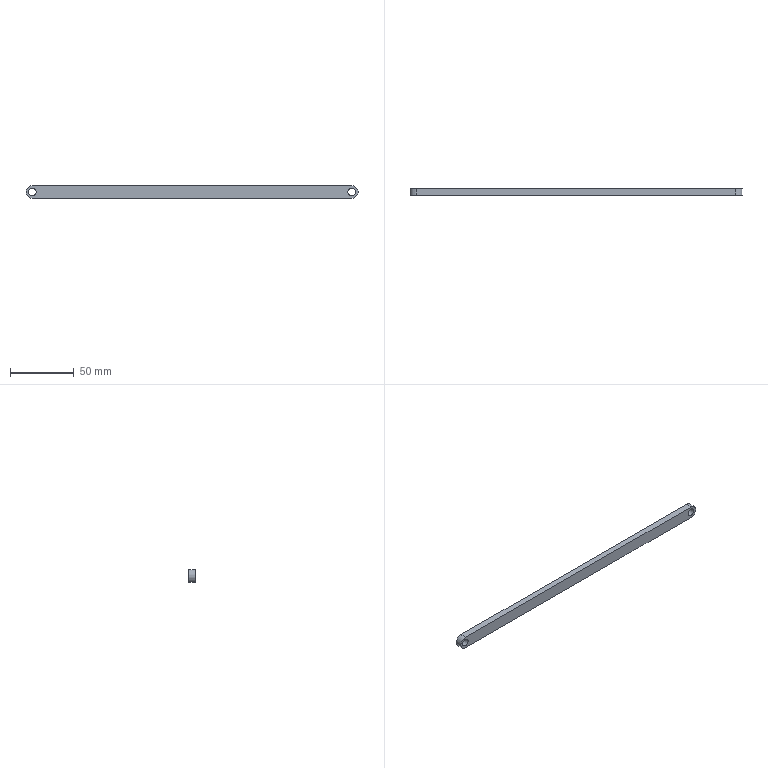Component | NX | 250 | 1 solid | 8 faces | box 260 x 5 x 10 mm | volume 12617 mm3 | plane 4 | cylinder 4 | commonest cylinder face diameters 10 x2 5.929 x2
STEP:
#1=CARTESIAN_POINT('',(0.,0.,0.));
#2=DIRECTION('',(0.,0.,1.));
#3=DIRECTION('',(1.,0.,0.));
#4=AXIS2_PLACEMENT_3D('',#1,#2,#3);
#5=CARTESIAN_POINT('',(-504.719,50.95,64.918));
#6=VERTEX_POINT('',#5);
#7=CARTESIAN_POINT('',(-254.719,50.95,64.918));
#8=VERTEX_POINT('',#7);
#9=CARTESIAN_POINT('',(-504.719,50.95,64.918));
#10=DIRECTION('',(1.,0.,-0.));
#11=VECTOR('',#10,1.);
#12=LINE('',#9,#11);
#13=CARTESIAN_POINT('',(-504.719,45.95,64.918));
#14=DIRECTION('',(0.,0.,1.));
#15=DIRECTION('',(1.,0.,-0.));
#16=AXIS2_PLACEMENT_3D('',#13,#14,#15);
#17=PLANE('',#16);
#18=CARTESIAN_POINT('',(0.,5.));
#19=DIRECTION('',(1.,0.));
#20=VECTOR('',#19,1.);
#21=LINE('',#18,#20);
#22=(GEOMETRIC_REPRESENTATION_CONTEXT(2)PARAMETRIC_REPRESENTATION_CONTEXT()REPRESENTATION_CONTEXT('',''));
#23=DEFINITIONAL_REPRESENTATION('',(#21),#22);
#24=PCURVE('',#17,#23);
#25=CARTESIAN_POINT('',(-254.719,50.95,59.918));
#26=DIRECTION('',(0.,1.,0.));
#27=DIRECTION('',(0.,0.,1.));
#28=AXIS2_PLACEMENT_3D('',#25,#26,#27);
#29=PLANE('',#28);
#30=CARTESIAN_POINT('',(5.,-250.));
#31=DIRECTION('',(-0.,1.));
#32=VECTOR('',#31,1.);
#33=LINE('',#30,#32);
#34=(GEOMETRIC_REPRESENTATION_CONTEXT(2)PARAMETRIC_REPRESENTATION_CONTEXT()REPRESENTATION_CONTEXT('',''));
#35=DEFINITIONAL_REPRESENTATION('',(#33),#34);
#36=PCURVE('',#29,#35);
#37=SURFACE_CURVE('',#12,(#24,#36),.PCURVE_S1.);
#38=EDGE_CURVE('',#6,#8,#37,.T.);
#39=ORIENTED_EDGE('',*,*,#38,.F.);
#40=CARTESIAN_POINT('',(-504.719,45.95,64.918));
#41=VERTEX_POINT('',#40);
#42=CARTESIAN_POINT('',(-504.719,45.95,64.918));
#43=DIRECTION('',(0.,1.,0.));
#44=VECTOR('',#43,1.);
#45=LINE('',#42,#44);
#46=CARTESIAN_POINT('',(0.,0.));
#47=DIRECTION('',(0.,1.));
#48=VECTOR('',#47,1.);
#49=LINE('',#46,#48);
#50=(GEOMETRIC_REPRESENTATION_CONTEXT(2)PARAMETRIC_REPRESENTATION_CONTEXT()REPRESENTATION_CONTEXT('',''));
#51=DEFINITIONAL_REPRESENTATION('',(#49),#50);
#52=PCURVE('',#17,#51);
#53=CARTESIAN_POINT('',(-504.719,45.95,59.918));
#54=DIRECTION('',(0.,1.,0.));
#55=DIRECTION('',(0.,0.,1.));
#56=AXIS2_PLACEMENT_3D('',#53,#54,#55);
#57=CYLINDRICAL_SURFACE('',#56,5.);
#58=CARTESIAN_POINT('',(6.283,0.));
#59=DIRECTION('',(0.,1.));
#60=VECTOR('',#59,1.);
#61=LINE('',#58,#60);
#62=(GEOMETRIC_REPRESENTATION_CONTEXT(2)PARAMETRIC_REPRESENTATION_CONTEXT()REPRESENTATION_CONTEXT('',''));
#63=DEFINITIONAL_REPRESENTATION('',(#61),#62);
#64=PCURVE('',#57,#63);
#65=SURFACE_CURVE('',#45,(#52,#64),.PCURVE_S1.);
#66=EDGE_CURVE('',#41,#6,#65,.T.);
#67=ORIENTED_EDGE('',*,*,#66,.F.);
#68=CARTESIAN_POINT('',(-254.719,45.95,64.918));
#69=VERTEX_POINT('',#68);
#70=CARTESIAN_POINT('',(-504.719,45.95,64.918));
#71=DIRECTION('',(1.,0.,-0.));
#72=VECTOR('',#71,1.);
#73=LINE('',#70,#72);
#74=CARTESIAN_POINT('',(0.,0.));
#75=DIRECTION('',(1.,0.));
#76=VECTOR('',#75,1.);
#77=LINE('',#74,#76);
#78=(GEOMETRIC_REPRESENTATION_CONTEXT(2)PARAMETRIC_REPRESENTATION_CONTEXT()REPRESENTATION_CONTEXT('',''));
#79=DEFINITIONAL_REPRESENTATION('',(#77),#78);
#80=PCURVE('',#17,#79);
#81=CARTESIAN_POINT('',(-254.719,45.95,59.918));
#82=DIRECTION('',(0.,1.,0.));
#83=DIRECTION('',(0.,0.,1.));
#84=AXIS2_PLACEMENT_3D('',#81,#82,#83);
#85=PLANE('',#84);
#86=CARTESIAN_POINT('',(5.,-250.));
#87=DIRECTION('',(-0.,1.));
#88=VECTOR('',#87,1.);
#89=LINE('',#86,#88);
#90=(GEOMETRIC_REPRESENTATION_CONTEXT(2)PARAMETRIC_REPRESENTATION_CONTEXT()REPRESENTATION_CONTEXT('',''));
#91=DEFINITIONAL_REPRESENTATION('',(#89),#90);
#92=PCURVE('',#85,#91);
#93=SURFACE_CURVE('',#73,(#80,#92),.PCURVE_S1.);
#94=EDGE_CURVE('',#41,#69,#93,.T.);
#95=ORIENTED_EDGE('',*,*,#94,.T.);
#96=CARTESIAN_POINT('',(-254.719,45.95,64.918));
#97=DIRECTION('',(0.,1.,0.));
#98=VECTOR('',#97,1.);
#99=LINE('',#96,#98);
#100=CARTESIAN_POINT('',(250.,0.));
#101=DIRECTION('',(0.,1.));
#102=VECTOR('',#101,1.);
#103=LINE('',#100,#102);
#104=(GEOMETRIC_REPRESENTATION_CONTEXT(2)PARAMETRIC_REPRESENTATION_CONTEXT()REPRESENTATION_CONTEXT('',''));
#105=DEFINITIONAL_REPRESENTATION('',(#103),#104);
#106=PCURVE('',#17,#105);
#107=CARTESIAN_POINT('',(-254.719,45.95,59.918));
#108=DIRECTION('',(0.,1.,0.));
#109=DIRECTION('',(0.,0.,1.));
#110=AXIS2_PLACEMENT_3D('',#107,#108,#109);
#111=CYLINDRICAL_SURFACE('',#110,5.);
#112=CARTESIAN_POINT('',(0.,0.));
#113=DIRECTION('',(0.,1.));
#114=VECTOR('',#113,1.);
#115=LINE('',#112,#114);
#116=(GEOMETRIC_REPRESENTATION_CONTEXT(2)PARAMETRIC_REPRESENTATION_CONTEXT()REPRESENTATION_CONTEXT('',''));
#117=DEFINITIONAL_REPRESENTATION('',(#115),#116);
#118=PCURVE('',#111,#117);
#119=SURFACE_CURVE('',#99,(#106,#118),.PCURVE_S1.);
#120=EDGE_CURVE('',#69,#8,#119,.T.);
#121=ORIENTED_EDGE('',*,*,#120,.T.);
#122=EDGE_LOOP('',(#39,#67,#95,#121));
#123=FACE_BOUND('',#122,.T.);
#124=ADVANCED_FACE('',(#123),#17,.T.);
#125=CARTESIAN_POINT('',(-254.719,50.95,54.918));
#126=VERTEX_POINT('',#125);
#127=CARTESIAN_POINT('',(-254.719,50.95,59.918));
#128=DIRECTION('',(0.,1.,0.));
#129=DIRECTION('',(0.,0.,1.));
#130=AXIS2_PLACEMENT_3D('',#127,#128,#129);
#131=CIRCLE('',#130,5.);
#132=CARTESIAN_POINT('',(0.,5.));
#133=DIRECTION('',(1.,0.));
#134=VECTOR('',#133,1.);
#135=LINE('',#132,#134);
#136=(GEOMETRIC_REPRESENTATION_CONTEXT(2)PARAMETRIC_REPRESENTATION_CONTEXT()REPRESENTATION_CONTEXT('',''));
#137=DEFINITIONAL_REPRESENTATION('',(#135),#136);
#138=PCURVE('',#111,#137);
#139=CARTESIAN_POINT('',(0.,0.));
#140=DIRECTION('',(1.,0.));
#141=AXIS2_PLACEMENT_2D('',#139,#140);
#142=CIRCLE('',#141,5.);
#143=(GEOMETRIC_REPRESENTATION_CONTEXT(2)PARAMETRIC_REPRESENTATION_CONTEXT()REPRESENTATION_CONTEXT('',''));
#144=DEFINITIONAL_REPRESENTATION('',(#142),#143);
#145=PCURVE('',#29,#144);
#146=SURFACE_CURVE('',#131,(#138,#145),.PCURVE_S1.);
#147=EDGE_CURVE('',#8,#126,#146,.T.);
#148=ORIENTED_EDGE('',*,*,#147,.F.);
#149=ORIENTED_EDGE('',*,*,#120,.F.);
#150=CARTESIAN_POINT('',(-254.719,45.95,54.918));
#151=VERTEX_POINT('',#150);
#152=CARTESIAN_POINT('',(-254.719,45.95,59.918));
#153=DIRECTION('',(0.,1.,0.));
#154=DIRECTION('',(0.,0.,1.));
#155=AXIS2_PLACEMENT_3D('',#152,#153,#154);
#156=CIRCLE('',#155,5.);
#157=CARTESIAN_POINT('',(0.,0.));
#158=DIRECTION('',(1.,0.));
#159=VECTOR('',#158,1.);
#160=LINE('',#157,#159);
#161=(GEOMETRIC_REPRESENTATION_CONTEXT(2)PARAMETRIC_REPRESENTATION_CONTEXT()REPRESENTATION_CONTEXT('',''));
#162=DEFINITIONAL_REPRESENTATION('',(#160),#161);
#163=PCURVE('',#111,#162);
#164=CARTESIAN_POINT('',(0.,0.));
#165=DIRECTION('',(1.,0.));
#166=AXIS2_PLACEMENT_2D('',#164,#165);
#167=CIRCLE('',#166,5.);
#168=(GEOMETRIC_REPRESENTATION_CONTEXT(2)PARAMETRIC_REPRESENTATION_CONTEXT()REPRESENTATION_CONTEXT('',''));
#169=DEFINITIONAL_REPRESENTATION('',(#167),#168);
#170=PCURVE('',#85,#169);
#171=SURFACE_CURVE('',#156,(#163,#170),.PCURVE_S1.);
#172=EDGE_CURVE('',#69,#151,#171,.T.);
#173=ORIENTED_EDGE('',*,*,#172,.T.);
#174=CARTESIAN_POINT('',(-254.719,45.95,54.918));
#175=DIRECTION('',(0.,1.,0.));
#176=VECTOR('',#175,1.);
#177=LINE('',#174,#176);
#178=CARTESIAN_POINT('',(3.142,0.));
#179=DIRECTION('',(0.,1.));
#180=VECTOR('',#179,1.);
#181=LINE('',#178,#180);
#182=(GEOMETRIC_REPRESENTATION_CONTEXT(2)PARAMETRIC_REPRESENTATION_CONTEXT()REPRESENTATION_CONTEXT('',''));
#183=DEFINITIONAL_REPRESENTATION('',(#181),#182);
#184=PCURVE('',#111,#183);
#185=CARTESIAN_POINT('',(-254.719,45.95,54.918));
#186=DIRECTION('',(0.,0.,-1.));
#187=DIRECTION('',(-1.,0.,-0.));
#188=AXIS2_PLACEMENT_3D('',#185,#186,#187);
#189=PLANE('',#188);
#190=CARTESIAN_POINT('',(0.,0.));
#191=DIRECTION('',(0.,1.));
#192=VECTOR('',#191,1.);
#193=LINE('',#190,#192);
#194=(GEOMETRIC_REPRESENTATION_CONTEXT(2)PARAMETRIC_REPRESENTATION_CONTEXT()REPRESENTATION_CONTEXT('',''));
#195=DEFINITIONAL_REPRESENTATION('',(#193),#194);
#196=PCURVE('',#189,#195);
#197=SURFACE_CURVE('',#177,(#184,#196),.PCURVE_S1.);
#198=EDGE_CURVE('',#151,#126,#197,.T.);
#199=ORIENTED_EDGE('',*,*,#198,.T.);
#200=EDGE_LOOP('',(#148,#149,#173,#199));
#201=FACE_BOUND('',#200,.T.);
#202=ADVANCED_FACE('',(#201),#111,.T.);
#203=CARTESIAN_POINT('',(-504.719,50.95,54.918));
#204=VERTEX_POINT('',#203);
#205=CARTESIAN_POINT('',(-254.719,50.95,54.918));
#206=DIRECTION('',(-1.,0.,-0.));
#207=VECTOR('',#206,1.);
#208=LINE('',#205,#207);
#209=CARTESIAN_POINT('',(0.,5.));
#210=DIRECTION('',(1.,0.));
#211=VECTOR('',#210,1.);
#212=LINE('',#209,#211);
#213=(GEOMETRIC_REPRESENTATION_CONTEXT(2)PARAMETRIC_REPRESENTATION_CONTEXT()REPRESENTATION_CONTEXT('',''));
#214=DEFINITIONAL_REPRESENTATION('',(#212),#213);
#215=PCURVE('',#189,#214);
#216=CARTESIAN_POINT('',(-5.,0.));
#217=DIRECTION('',(-0.,-1.));
#218=VECTOR('',#217,1.);
#219=LINE('',#216,#218);
#220=(GEOMETRIC_REPRESENTATION_CONTEXT(2)PARAMETRIC_REPRESENTATION_CONTEXT()REPRESENTATION_CONTEXT('',''));
#221=DEFINITIONAL_REPRESENTATION('',(#219),#220);
#222=PCURVE('',#29,#221);
#223=SURFACE_CURVE('',#208,(#215,#222),.PCURVE_S1.);
#224=EDGE_CURVE('',#126,#204,#223,.T.);
#225=ORIENTED_EDGE('',*,*,#224,.F.);
#226=ORIENTED_EDGE('',*,*,#198,.F.);
#227=CARTESIAN_POINT('',(-504.719,45.95,54.918));
#228=VERTEX_POINT('',#227);
#229=CARTESIAN_POINT('',(-254.719,45.95,54.918));
#230=DIRECTION('',(-1.,0.,-0.));
#231=VECTOR('',#230,1.);
#232=LINE('',#229,#231);
#233=CARTESIAN_POINT('',(0.,0.));
#234=DIRECTION('',(1.,0.));
#235=VECTOR('',#234,1.);
#236=LINE('',#233,#235);
#237=(GEOMETRIC_REPRESENTATION_CONTEXT(2)PARAMETRIC_REPRESENTATION_CONTEXT()REPRESENTATION_CONTEXT('',''));
#238=DEFINITIONAL_REPRESENTATION('',(#236),#237);
#239=PCURVE('',#189,#238);
#240=CARTESIAN_POINT('',(-5.,0.));
#241=DIRECTION('',(-0.,-1.));
#242=VECTOR('',#241,1.);
#243=LINE('',#240,#242);
#244=(GEOMETRIC_REPRESENTATION_CONTEXT(2)PARAMETRIC_REPRESENTATION_CONTEXT()REPRESENTATION_CONTEXT('',''));
#245=DEFINITIONAL_REPRESENTATION('',(#243),#244);
#246=PCURVE('',#85,#245);
#247=SURFACE_CURVE('',#232,(#239,#246),.PCURVE_S1.);
#248=EDGE_CURVE('',#151,#228,#247,.T.);
#249=ORIENTED_EDGE('',*,*,#248,.T.);
#250=CARTESIAN_POINT('',(-504.719,45.95,54.918));
#251=DIRECTION('',(0.,1.,0.));
#252=VECTOR('',#251,1.);
#253=LINE('',#250,#252);
#254=CARTESIAN_POINT('',(250.,0.));
#255=DIRECTION('',(0.,1.));
#256=VECTOR('',#255,1.);
#257=LINE('',#254,#256);
#258=(GEOMETRIC_REPRESENTATION_CONTEXT(2)PARAMETRIC_REPRESENTATION_CONTEXT()REPRESENTATION_CONTEXT('',''));
#259=DEFINITIONAL_REPRESENTATION('',(#257),#258);
#260=PCURVE('',#189,#259);
#261=CARTESIAN_POINT('',(3.142,0.));
#262=DIRECTION('',(0.,1.));
#263=VECTOR('',#262,1.);
#264=LINE('',#261,#263);
#265=(GEOMETRIC_REPRESENTATION_CONTEXT(2)PARAMETRIC_REPRESENTATION_CONTEXT()REPRESENTATION_CONTEXT('',''));
#266=DEFINITIONAL_REPRESENTATION('',(#264),#265);
#267=PCURVE('',#57,#266);
#268=SURFACE_CURVE('',#253,(#260,#267),.PCURVE_S1.);
#269=EDGE_CURVE('',#228,#204,#268,.T.);
#270=ORIENTED_EDGE('',*,*,#269,.T.);
#271=EDGE_LOOP('',(#225,#226,#249,#270));
#272=FACE_BOUND('',#271,.T.);
#273=ADVANCED_FACE('',(#272),#189,.T.);
#274=CARTESIAN_POINT('',(-504.719,45.95,62.883));
#275=VERTEX_POINT('',#274);
#276=CARTESIAN_POINT('',(-504.719,45.95,59.918));
#277=DIRECTION('',(0.,1.,0.));
#278=DIRECTION('',(0.,0.,1.));
#279=AXIS2_PLACEMENT_3D('',#276,#277,#278);
#280=CIRCLE('',#279,2.964);
#281=CARTESIAN_POINT('',(-504.719,45.95,59.918));
#282=DIRECTION('',(0.,1.,0.));
#283=DIRECTION('',(0.,0.,1.));
#284=AXIS2_PLACEMENT_3D('',#281,#282,#283);
#285=CYLINDRICAL_SURFACE('',#284,2.964);
#286=CARTESIAN_POINT('',(0.,0.));
#287=DIRECTION('',(1.,0.));
#288=VECTOR('',#287,1.);
#289=LINE('',#286,#288);
#290=(GEOMETRIC_REPRESENTATION_CONTEXT(2)PARAMETRIC_REPRESENTATION_CONTEXT()REPRESENTATION_CONTEXT('',''));
#291=DEFINITIONAL_REPRESENTATION('',(#289),#290);
#292=PCURVE('',#285,#291);
#293=CARTESIAN_POINT('',(0.,-250.));
#294=DIRECTION('',(1.,0.));
#295=AXIS2_PLACEMENT_2D('',#293,#294);
#296=CIRCLE('',#295,2.964);
#297=(GEOMETRIC_REPRESENTATION_CONTEXT(2)PARAMETRIC_REPRESENTATION_CONTEXT()REPRESENTATION_CONTEXT('',''));
#298=DEFINITIONAL_REPRESENTATION('',(#296),#297);
#299=PCURVE('',#85,#298);
#300=SURFACE_CURVE('',#280,(#292,#299),.PCURVE_S1.);
#301=EDGE_CURVE('',#275,#275,#300,.T.);
#302=ORIENTED_EDGE('',*,*,#301,.T.);
#303=CARTESIAN_POINT('',(-504.719,50.95,62.883));
#304=VERTEX_POINT('',#303);
#305=CARTESIAN_POINT('',(-504.719,45.95,62.883));
#306=CARTESIAN_POINT('',(-504.719,50.95,62.883));
#307=B_SPLINE_CURVE_WITH_KNOTS('',1,(#305,#306),.UNSPECIFIED.,.F.,.F.,(2,2),(0.,5.),.PIECEWISE_BEZIER_KNOTS.);
#308=CARTESIAN_POINT('',(6.283,0.));
#309=DIRECTION('',(0.,1.));
#310=VECTOR('',#309,1.);
#311=LINE('',#308,#310);
#312=(GEOMETRIC_REPRESENTATION_CONTEXT(2)PARAMETRIC_REPRESENTATION_CONTEXT()REPRESENTATION_CONTEXT('',''));
#313=DEFINITIONAL_REPRESENTATION('',(#311),#312);
#314=PCURVE('',#285,#313);
#315=CARTESIAN_POINT('',(0.,0.));
#316=DIRECTION('',(0.,1.));
#317=VECTOR('',#316,1.);
#318=LINE('',#315,#317);
#319=(GEOMETRIC_REPRESENTATION_CONTEXT(2)PARAMETRIC_REPRESENTATION_CONTEXT()REPRESENTATION_CONTEXT('',''));
#320=DEFINITIONAL_REPRESENTATION('',(#318),#319);
#321=PCURVE('',#285,#320);
#322=SEAM_CURVE('',#307,(#314,#321),.PCURVE_S1.);
#323=EDGE_CURVE('',#275,#304,#322,.T.);
#324=ORIENTED_EDGE('',*,*,#323,.T.);
#325=CARTESIAN_POINT('',(-504.719,50.95,59.918));
#326=DIRECTION('',(0.,1.,0.));
#327=DIRECTION('',(0.,0.,1.));
#328=AXIS2_PLACEMENT_3D('',#325,#326,#327);
#329=CIRCLE('',#328,2.964);
#330=CARTESIAN_POINT('',(0.,5.));
#331=DIRECTION('',(1.,0.));
#332=VECTOR('',#331,1.);
#333=LINE('',#330,#332);
#334=(GEOMETRIC_REPRESENTATION_CONTEXT(2)PARAMETRIC_REPRESENTATION_CONTEXT()REPRESENTATION_CONTEXT('',''));
#335=DEFINITIONAL_REPRESENTATION('',(#333),#334);
#336=PCURVE('',#285,#335);
#337=CARTESIAN_POINT('',(0.,-250.));
#338=DIRECTION('',(1.,0.));
#339=AXIS2_PLACEMENT_2D('',#337,#338);
#340=CIRCLE('',#339,2.964);
#341=(GEOMETRIC_REPRESENTATION_CONTEXT(2)PARAMETRIC_REPRESENTATION_CONTEXT()REPRESENTATION_CONTEXT('',''));
#342=DEFINITIONAL_REPRESENTATION('',(#340),#341);
#343=PCURVE('',#29,#342);
#344=SURFACE_CURVE('',#329,(#336,#343),.PCURVE_S1.);
#345=EDGE_CURVE('',#304,#304,#344,.T.);
#346=ORIENTED_EDGE('',*,*,#345,.F.);
#347=ORIENTED_EDGE('',*,*,#323,.F.);
#348=EDGE_LOOP('',(#302,#324,#346,#347));
#349=FACE_BOUND('',#348,.F.);
#350=ADVANCED_FACE('',(#349),#285,.F.);
#351=CARTESIAN_POINT('',(-504.719,50.95,59.918));
#352=DIRECTION('',(0.,1.,0.));
#353=DIRECTION('',(0.,0.,1.));
#354=AXIS2_PLACEMENT_3D('',#351,#352,#353);
#355=CIRCLE('',#354,5.);
#356=CARTESIAN_POINT('',(0.,5.));
#357=DIRECTION('',(1.,0.));
#358=VECTOR('',#357,1.);
#359=LINE('',#356,#358);
#360=(GEOMETRIC_REPRESENTATION_CONTEXT(2)PARAMETRIC_REPRESENTATION_CONTEXT()REPRESENTATION_CONTEXT('',''));
#361=DEFINITIONAL_REPRESENTATION('',(#359),#360);
#362=PCURVE('',#57,#361);
#363=CARTESIAN_POINT('',(0.,-250.));
#364=DIRECTION('',(1.,0.));
#365=AXIS2_PLACEMENT_2D('',#363,#364);
#366=CIRCLE('',#365,5.);
#367=(GEOMETRIC_REPRESENTATION_CONTEXT(2)PARAMETRIC_REPRESENTATION_CONTEXT()REPRESENTATION_CONTEXT('',''));
#368=DEFINITIONAL_REPRESENTATION('',(#366),#367);
#369=PCURVE('',#29,#368);
#370=SURFACE_CURVE('',#355,(#362,#369),.PCURVE_S1.);
#371=EDGE_CURVE('',#204,#6,#370,.T.);
#372=ORIENTED_EDGE('',*,*,#371,.F.);
#373=ORIENTED_EDGE('',*,*,#269,.F.);
#374=CARTESIAN_POINT('',(-504.719,45.95,59.918));
#375=DIRECTION('',(0.,1.,0.));
#376=DIRECTION('',(0.,0.,1.));
#377=AXIS2_PLACEMENT_3D('',#374,#375,#376);
#378=CIRCLE('',#377,5.);
#379=CARTESIAN_POINT('',(0.,0.));
#380=DIRECTION('',(1.,0.));
#381=VECTOR('',#380,1.);
#382=LINE('',#379,#381);
#383=(GEOMETRIC_REPRESENTATION_CONTEXT(2)PARAMETRIC_REPRESENTATION_CONTEXT()REPRESENTATION_CONTEXT('',''));
#384=DEFINITIONAL_REPRESENTATION('',(#382),#383);
#385=PCURVE('',#57,#384);
#386=CARTESIAN_POINT('',(0.,-250.));
#387=DIRECTION('',(1.,0.));
#388=AXIS2_PLACEMENT_2D('',#386,#387);
#389=CIRCLE('',#388,5.);
#390=(GEOMETRIC_REPRESENTATION_CONTEXT(2)PARAMETRIC_REPRESENTATION_CONTEXT()REPRESENTATION_CONTEXT('',''));
#391=DEFINITIONAL_REPRESENTATION('',(#389),#390);
#392=PCURVE('',#85,#391);
#393=SURFACE_CURVE('',#378,(#385,#392),.PCURVE_S1.);
#394=EDGE_CURVE('',#228,#41,#393,.T.);
#395=ORIENTED_EDGE('',*,*,#394,.T.);
#396=ORIENTED_EDGE('',*,*,#66,.T.);
#397=EDGE_LOOP('',(#372,#373,#395,#396));
#398=FACE_BOUND('',#397,.T.);
#399=ADVANCED_FACE('',(#398),#57,.T.);
#400=CARTESIAN_POINT('',(-254.719,45.95,62.883));
#401=VERTEX_POINT('',#400);
#402=CARTESIAN_POINT('',(-254.719,45.95,59.918));
#403=DIRECTION('',(0.,1.,0.));
#404=DIRECTION('',(0.,0.,1.));
#405=AXIS2_PLACEMENT_3D('',#402,#403,#404);
#406=CIRCLE('',#405,2.964);
#407=CARTESIAN_POINT('',(-254.719,45.95,59.918));
#408=DIRECTION('',(0.,1.,0.));
#409=DIRECTION('',(0.,0.,1.));
#410=AXIS2_PLACEMENT_3D('',#407,#408,#409);
#411=CYLINDRICAL_SURFACE('',#410,2.964);
#412=CARTESIAN_POINT('',(0.,0.));
#413=DIRECTION('',(1.,0.));
#414=VECTOR('',#413,1.);
#415=LINE('',#412,#414);
#416=(GEOMETRIC_REPRESENTATION_CONTEXT(2)PARAMETRIC_REPRESENTATION_CONTEXT()REPRESENTATION_CONTEXT('',''));
#417=DEFINITIONAL_REPRESENTATION('',(#415),#416);
#418=PCURVE('',#411,#417);
#419=CARTESIAN_POINT('',(0.,0.));
#420=DIRECTION('',(1.,0.));
#421=AXIS2_PLACEMENT_2D('',#419,#420);
#422=CIRCLE('',#421,2.964);
#423=(GEOMETRIC_REPRESENTATION_CONTEXT(2)PARAMETRIC_REPRESENTATION_CONTEXT()REPRESENTATION_CONTEXT('',''));
#424=DEFINITIONAL_REPRESENTATION('',(#422),#423);
#425=PCURVE('',#85,#424);
#426=SURFACE_CURVE('',#406,(#418,#425),.PCURVE_S1.);
#427=EDGE_CURVE('',#401,#401,#426,.T.);
#428=ORIENTED_EDGE('',*,*,#427,.T.);
#429=CARTESIAN_POINT('',(-254.719,50.95,62.883));
#430=VERTEX_POINT('',#429);
#431=CARTESIAN_POINT('',(-254.719,45.95,62.883));
#432=CARTESIAN_POINT('',(-254.719,50.95,62.883));
#433=B_SPLINE_CURVE_WITH_KNOTS('',1,(#431,#432),.UNSPECIFIED.,.F.,.F.,(2,2),(0.,5.),.PIECEWISE_BEZIER_KNOTS.);
#434=CARTESIAN_POINT('',(6.283,0.));
#435=DIRECTION('',(0.,1.));
#436=VECTOR('',#435,1.);
#437=LINE('',#434,#436);
#438=(GEOMETRIC_REPRESENTATION_CONTEXT(2)PARAMETRIC_REPRESENTATION_CONTEXT()REPRESENTATION_CONTEXT('',''));
#439=DEFINITIONAL_REPRESENTATION('',(#437),#438);
#440=PCURVE('',#411,#439);
#441=CARTESIAN_POINT('',(0.,0.));
#442=DIRECTION('',(0.,1.));
#443=VECTOR('',#442,1.);
#444=LINE('',#441,#443);
#445=(GEOMETRIC_REPRESENTATION_CONTEXT(2)PARAMETRIC_REPRESENTATION_CONTEXT()REPRESENTATION_CONTEXT('',''));
#446=DEFINITIONAL_REPRESENTATION('',(#444),#445);
#447=PCURVE('',#411,#446);
#448=SEAM_CURVE('',#433,(#440,#447),.PCURVE_S1.);
#449=EDGE_CURVE('',#401,#430,#448,.T.);
#450=ORIENTED_EDGE('',*,*,#449,.T.);
#451=CARTESIAN_POINT('',(-254.719,50.95,59.918));
#452=DIRECTION('',(0.,1.,0.));
#453=DIRECTION('',(0.,0.,1.));
#454=AXIS2_PLACEMENT_3D('',#451,#452,#453);
#455=CIRCLE('',#454,2.964);
#456=CARTESIAN_POINT('',(0.,5.));
#457=DIRECTION('',(1.,0.));
#458=VECTOR('',#457,1.);
#459=LINE('',#456,#458);
#460=(GEOMETRIC_REPRESENTATION_CONTEXT(2)PARAMETRIC_REPRESENTATION_CONTEXT()REPRESENTATION_CONTEXT('',''));
#461=DEFINITIONAL_REPRESENTATION('',(#459),#460);
#462=PCURVE('',#411,#461);
#463=CARTESIAN_POINT('',(0.,0.));
#464=DIRECTION('',(1.,0.));
#465=AXIS2_PLACEMENT_2D('',#463,#464);
#466=CIRCLE('',#465,2.964);
#467=(GEOMETRIC_REPRESENTATION_CONTEXT(2)PARAMETRIC_REPRESENTATION_CONTEXT()REPRESENTATION_CONTEXT('',''));
#468=DEFINITIONAL_REPRESENTATION('',(#466),#467);
#469=PCURVE('',#29,#468);
#470=SURFACE_CURVE('',#455,(#462,#469),.PCURVE_S1.);
#471=EDGE_CURVE('',#430,#430,#470,.T.);
#472=ORIENTED_EDGE('',*,*,#471,.F.);
#473=ORIENTED_EDGE('',*,*,#449,.F.);
#474=EDGE_LOOP('',(#428,#450,#472,#473));
#475=FACE_BOUND('',#474,.F.);
#476=ADVANCED_FACE('',(#475),#411,.F.);
#477=ORIENTED_EDGE('',*,*,#94,.F.);
#478=ORIENTED_EDGE('',*,*,#394,.F.);
#479=ORIENTED_EDGE('',*,*,#248,.F.);
#480=ORIENTED_EDGE('',*,*,#172,.F.);
#481=EDGE_LOOP('',(#477,#478,#479,#480));
#482=FACE_BOUND('',#481,.T.);
#483=ORIENTED_EDGE('',*,*,#301,.T.);
#484=EDGE_LOOP('',(#483));
#485=FACE_BOUND('',#484,.T.);
#486=ORIENTED_EDGE('',*,*,#427,.T.);
#487=EDGE_LOOP('',(#486));
#488=FACE_BOUND('',#487,.T.);
#489=ADVANCED_FACE('',(#482,#485,#488),#85,.F.);
#490=ORIENTED_EDGE('',*,*,#38,.T.);
#491=ORIENTED_EDGE('',*,*,#147,.T.);
#492=ORIENTED_EDGE('',*,*,#224,.T.);
#493=ORIENTED_EDGE('',*,*,#371,.T.);
#494=EDGE_LOOP('',(#490,#491,#492,#493));
#495=FACE_BOUND('',#494,.T.);
#496=ORIENTED_EDGE('',*,*,#345,.F.);
#497=EDGE_LOOP('',(#496));
#498=FACE_BOUND('',#497,.T.);
#499=ORIENTED_EDGE('',*,*,#471,.F.);
#500=EDGE_LOOP('',(#499));
#501=FACE_BOUND('',#500,.T.);
#502=ADVANCED_FACE('',(#495,#498,#501),#29,.T.);
#503=CLOSED_SHELL('',(#124,#202,#273,#350,#399,#476,#489,#502));
#504=MANIFOLD_SOLID_BREP('',#503);
#505=(LENGTH_UNIT()NAMED_UNIT(*)SI_UNIT(.MILLI.,.METRE.));
#506=UNCERTAINTY_MEASURE_WITH_UNIT(LENGTH_MEASURE(0.000002),#505,'','');
#507=(NAMED_UNIT(*)PLANE_ANGLE_UNIT()SI_UNIT($,.RADIAN.));
#508=(NAMED_UNIT(*)SI_UNIT($,.STERADIAN.)SOLID_ANGLE_UNIT());
#509=(GEOMETRIC_REPRESENTATION_CONTEXT(3)GLOBAL_UNCERTAINTY_ASSIGNED_CONTEXT((#506))GLOBAL_UNIT_ASSIGNED_CONTEXT((#505,#507,#508))REPRESENTATION_CONTEXT('',''));
#510=ADVANCED_BREP_SHAPE_REPRESENTATION('',(#4,#504),#509);